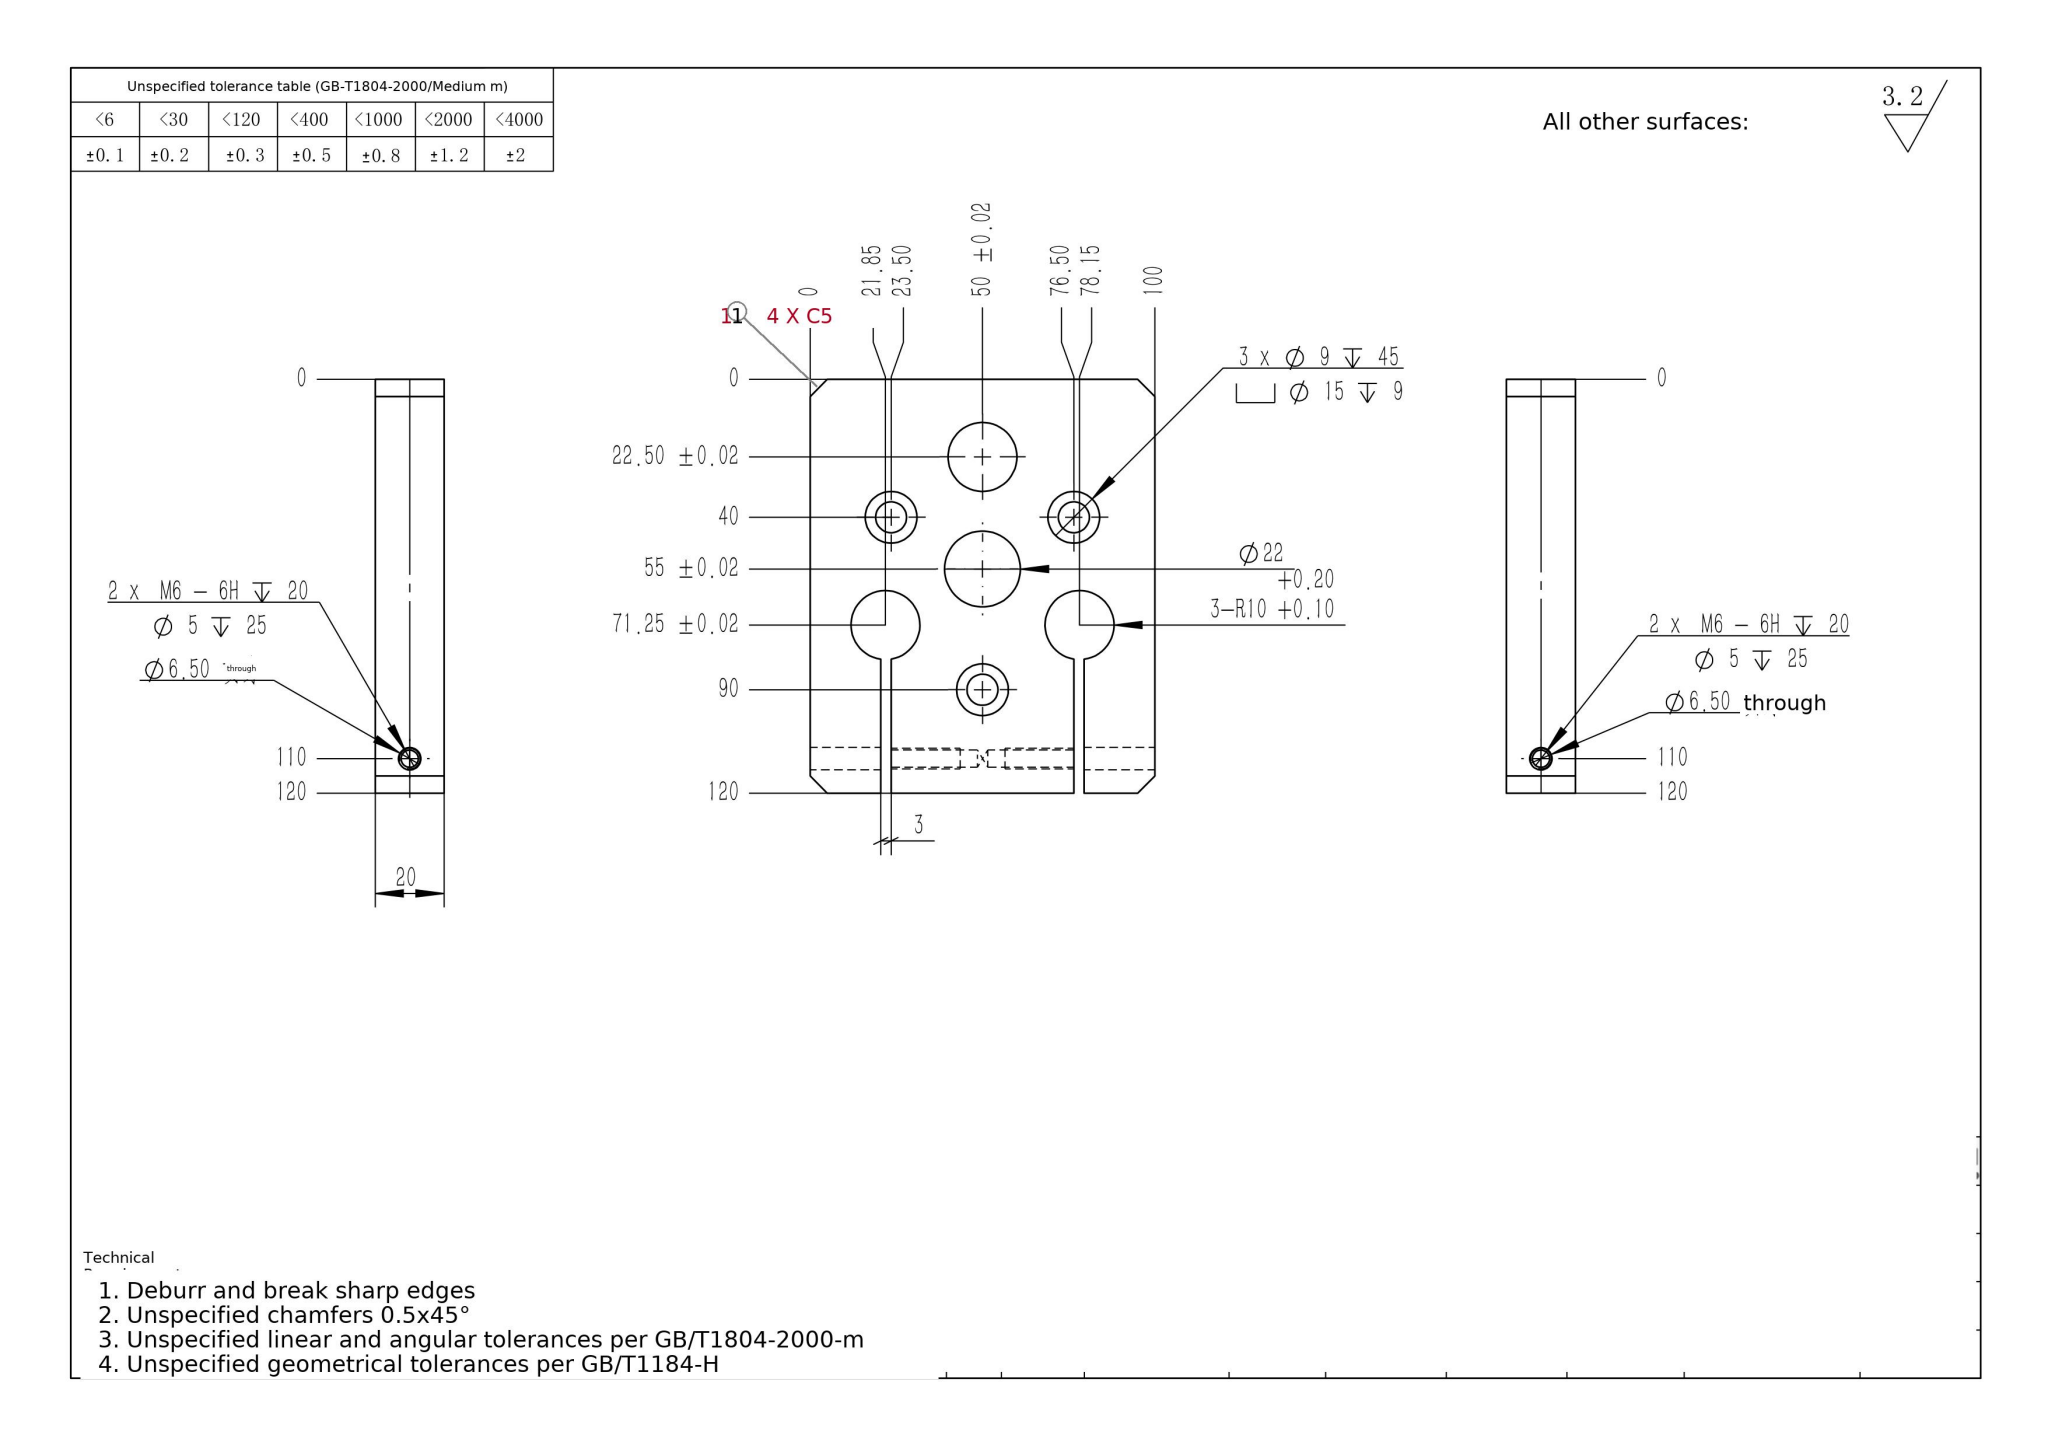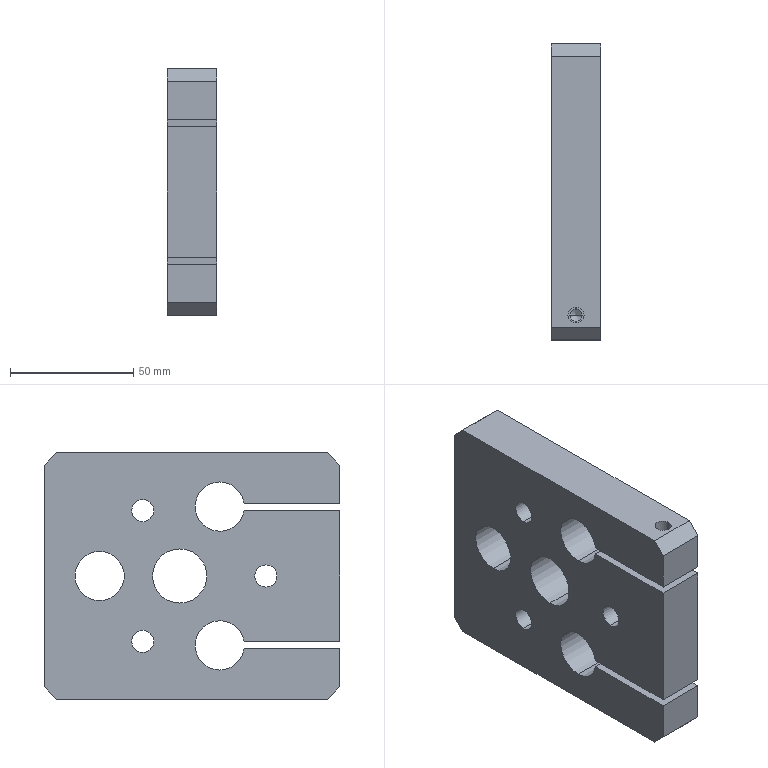Part | SolidWorks | mm | 1 solid | 53 faces | box 20 x 120 x 100 mm | volume 198661 mm3 | cylinder 30 | plane 19 | cone 4 | commonest cylinder face diameters 20 x8 15 x6 9 x6 5 x4 6.5 x4 22 x2
build123d program:
from build123d import *

# Parameters (mm, degrees)
SKETCH1_W                                         = 100
SKETCH1_H                                         = 120
BOSS_EXTRUDE1_DEPTH                               = 20
SKETCH2_R                                         = 10
SKETCH2_R_2                                       = 11
CUT_EXTRUDE1_DEPTH                                = 81.623
SKETCH3_W                                         = 3
SKETCH3_H                                         = 40
CUT_EXTRUDE2_DEPTH                                = 81.623
HOLE_SIZE_ACCORDING_TO_HEXAGON_SOCKET_D           = 9
HOLE_SIZE_ACCORDING_TO_HEXAGON_SOCKET_DEPTH       = 45
HOLE_SIZE_ACCORDING_TO_HEXAGON_SOCKET_CBORE_D     = 15
HOLE_SIZE_ACCORDING_TO_HEXAGON_SOCKET_CBORE_DEPTH = 9
HOLE_SIZE_ACCORDING_TO_HEXAGON_SOCKET_TIP         = 2.704
CUT_EXTRUDE3_REACH                                = 120.322
SKETCH6_R                                         = 3.25
CHAMFER1_SIZE                                     = 5


with BuildPart() as part:
    # Sketch1 → Boss-Extrude1 (new body)
    with BuildSketch(Plane(origin=(0, 0, 0), x_dir=(0, 0, -1), z_dir=(1, 0, 0))):
        Rectangle(SKETCH1_W, SKETCH1_H)
    extrude(amount=BOSS_EXTRUDE1_DEPTH)

    # Sketch2 → Cut-Extrude1 (cut, through all)
    with BuildSketch(Plane(origin=(20, 0, 0), x_dir=(0, 0, -1), z_dir=(1, 0, 0))):
        with Locations((0, 37.5)):
            Circle(SKETCH2_R)
        with Locations((0, 5)):
            Circle(SKETCH2_R_2)
        with Locations((28.146, -11.25)):
            Circle(SKETCH2_R)
        with Locations((-28.146, -11.25)):
            Circle(SKETCH2_R)
    extrude(amount=-CUT_EXTRUDE1_DEPTH, mode=Mode.SUBTRACT)

    # Sketch3 → Cut-Extrude2 (cut, through all)
    with BuildSketch(Plane.ZY):
        with Locations((-28, -40)):
            Rectangle(SKETCH3_W, SKETCH3_H)
        with Locations((28, -40)):
            Rectangle(SKETCH3_W, SKETCH3_H)
    extrude(amount=-CUT_EXTRUDE2_DEPTH, mode=Mode.SUBTRACT)

    # Hole Size _according to_ Hexagon Socket
    with Locations(Plane(origin=(20, 0, 0), x_dir=(0, 0, 1), z_dir=(1, 0, 0))):
        with Locations((-26.5, -20), (26.5, -20), (0, 30)):
            CounterBoreHole(HOLE_SIZE_ACCORDING_TO_HEXAGON_SOCKET_D / 2, HOLE_SIZE_ACCORDING_TO_HEXAGON_SOCKET_CBORE_D / 2, HOLE_SIZE_ACCORDING_TO_HEXAGON_SOCKET_CBORE_DEPTH, depth=HOLE_SIZE_ACCORDING_TO_HEXAGON_SOCKET_DEPTH)
            with Locations((0, 0, -(HOLE_SIZE_ACCORDING_TO_HEXAGON_SOCKET_DEPTH + HOLE_SIZE_ACCORDING_TO_HEXAGON_SOCKET_TIP / 2))):  # 118° drill point
                Cone(0, HOLE_SIZE_ACCORDING_TO_HEXAGON_SOCKET_D / 2, HOLE_SIZE_ACCORDING_TO_HEXAGON_SOCKET_TIP, mode=Mode.SUBTRACT)

    # Sketch6 → Cut-Extrude3 (cut, up to next)
    with BuildSketch(Plane.XY.offset(50), mode=Mode.PRIVATE) as cut_extrude3_sk1:
        with Locations((10, -50)):
            Circle(SKETCH6_R)
    cut_extrude3_tool1 = extrude(cut_extrude3_sk1.sketch, amount=-CUT_EXTRUDE3_REACH, mode=Mode.PRIVATE) & part.part
    cut_extrude3 = cut_extrude3_tool1.solids().sort_by_distance((10, -50, 50))[0]
    add(cut_extrude3, mode=Mode.SUBTRACT)

    # Sketch8 → M6 Tapped Hole1 (revolve, cut)
    with BuildSketch(Plane(origin=(10, -50, 26.5), x_dir=(0, -1, 0), z_dir=(1, 0, 0))):
        Polygon((0, 0), (0, 26.502), (2.5, 25), (2.5, 0), align=None)
    m6_tapped_hole1 = revolve(axis=Axis((10, -50, 32.85), (0, 0, -1)), mode=Mode.SUBTRACT)

    # Mirror1: Cut-Extrude3, M6 Tapped Hole1 across plane
    add(cut_extrude3.mirror(Plane.XY), mode=Mode.SUBTRACT)
    add(m6_tapped_hole1.mirror(Plane.XY), mode=Mode.SUBTRACT)

    # Chamfer1
    chamfer1_edges = [part.edges().sort_by_distance(p)[0] for p in [
        (10, -60, -50),
        (10, -60, 50),
        (10, 60, 50),
        (10, 60, -50),
    ]]
    chamfer(chamfer1_edges, length=CHAMFER1_SIZE)


solid = part.part